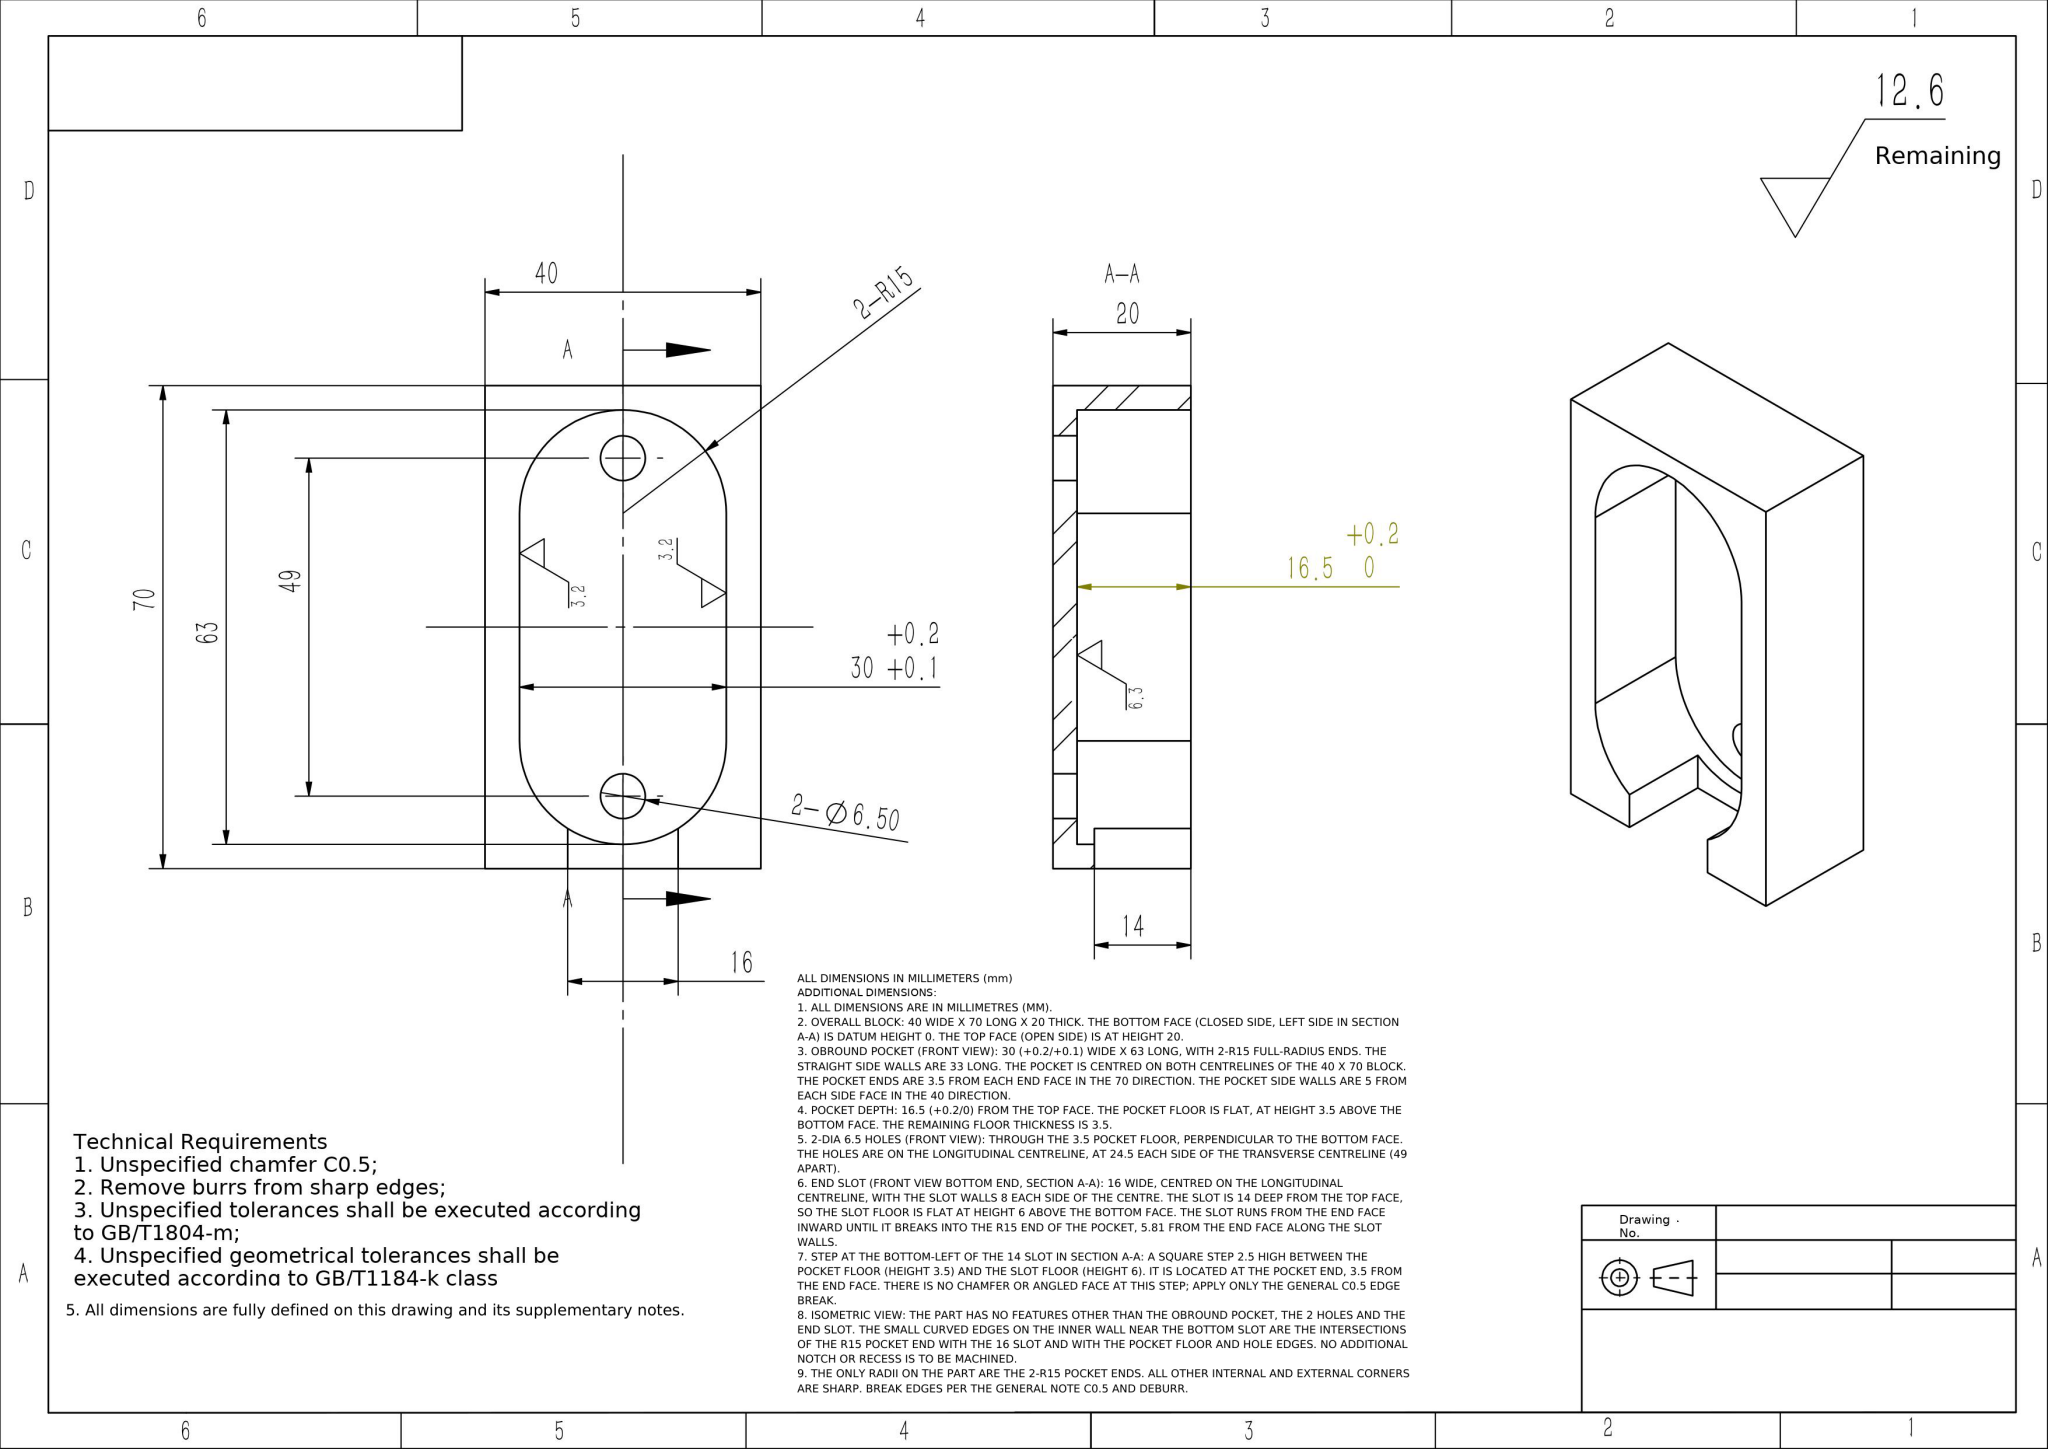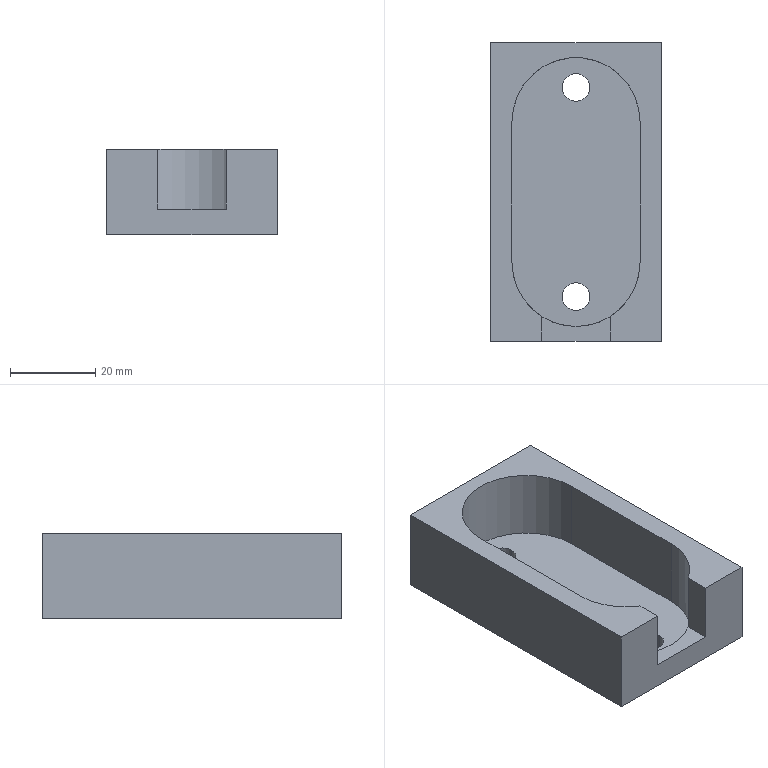Part | NX | mm | 1 solid | 18 faces | box 40 x 70 x 20 mm | volume 26819 mm3 | plane 12 | cylinder 6 | commonest cylinder face diameters 6.5 x4 30 x2